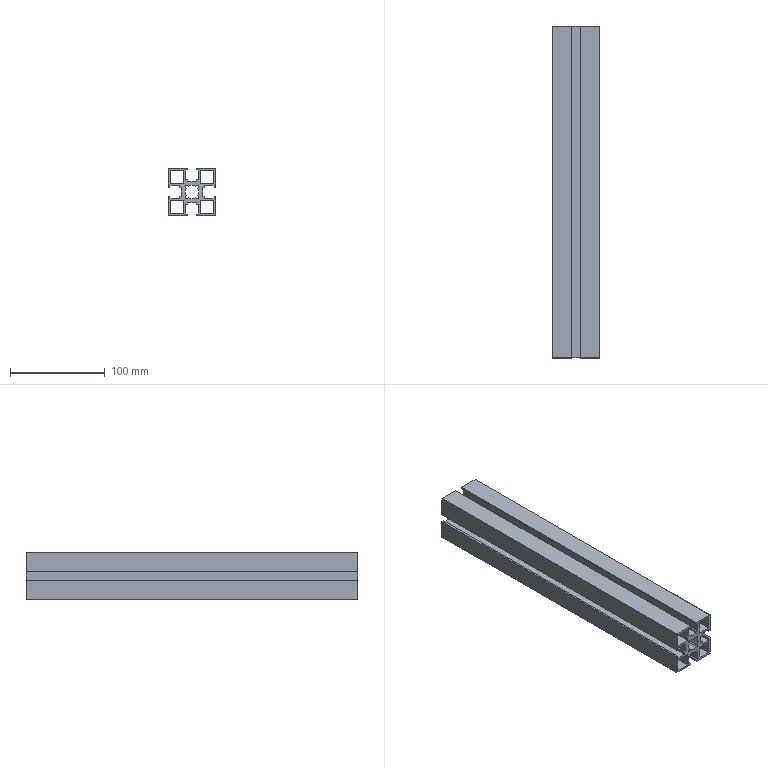CAM job | Mastercam | mm | 4 operations | part box 50 x 350 x 50
1. Contour (Ramp) | 16 - 16 平铣刀
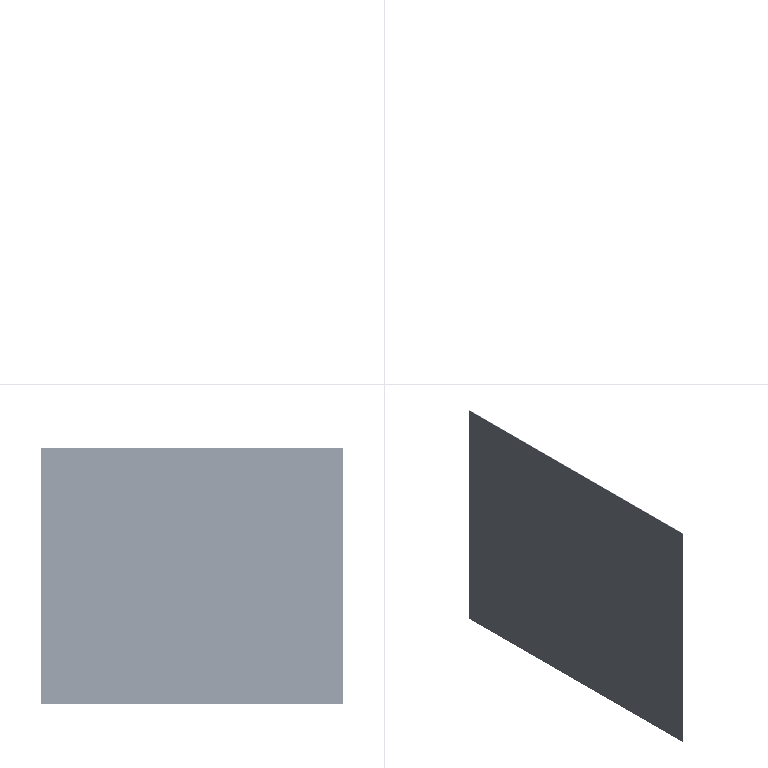2. Contour (2D) | 16 - 16 平铣刀
3. Contour (Ramp) | 16 - 16 平铣刀
4. Contour (2D) | 16 - 16 平铣刀